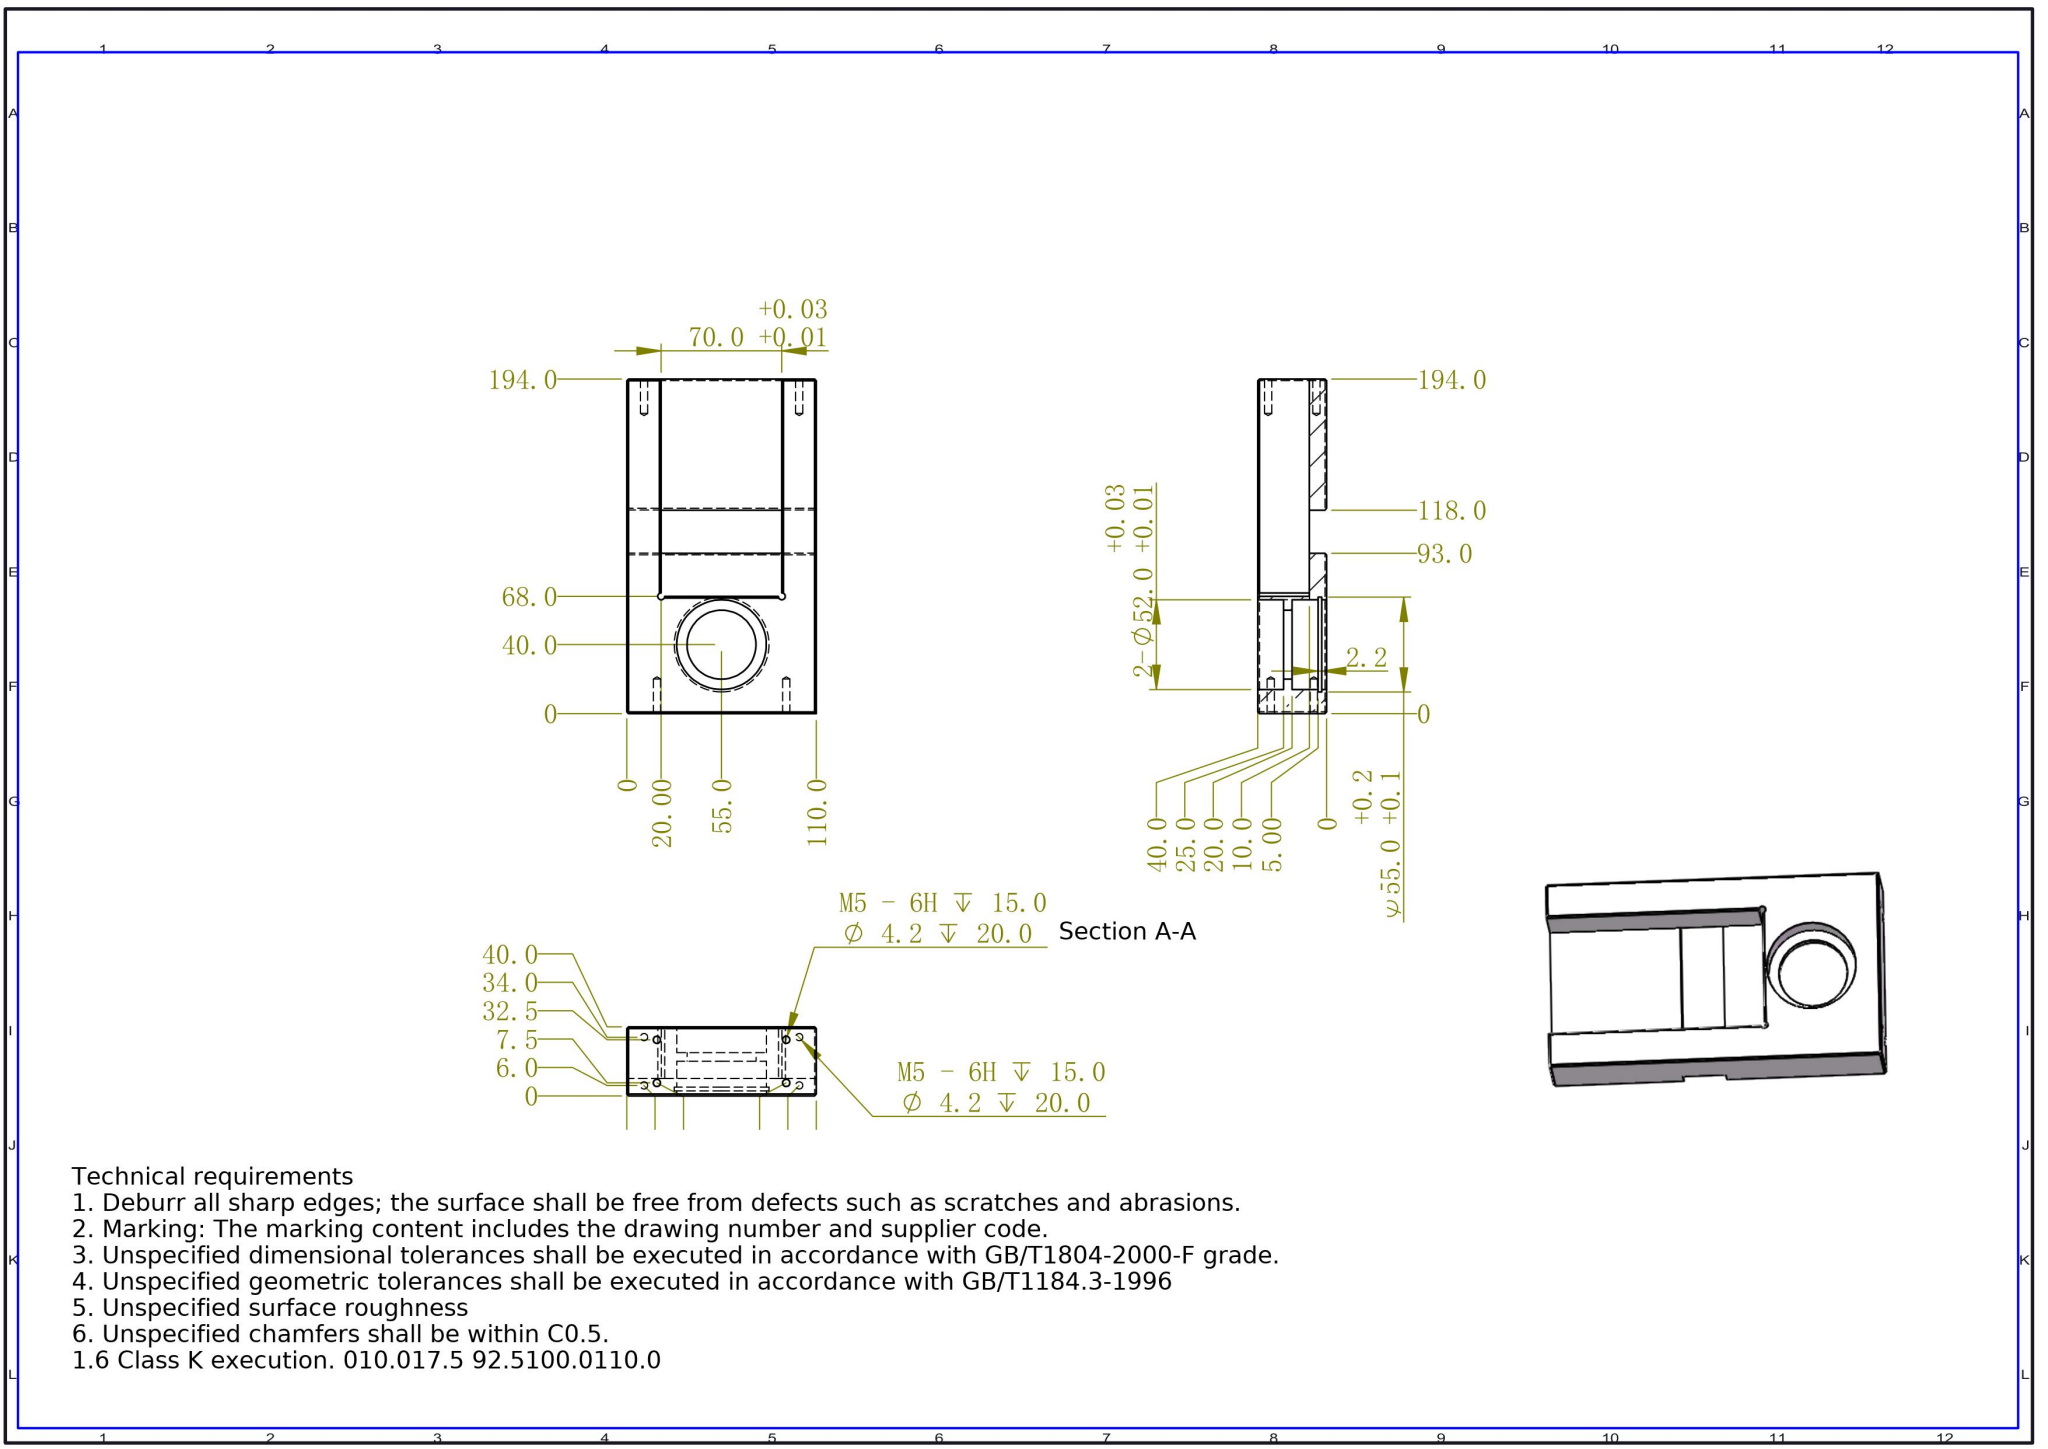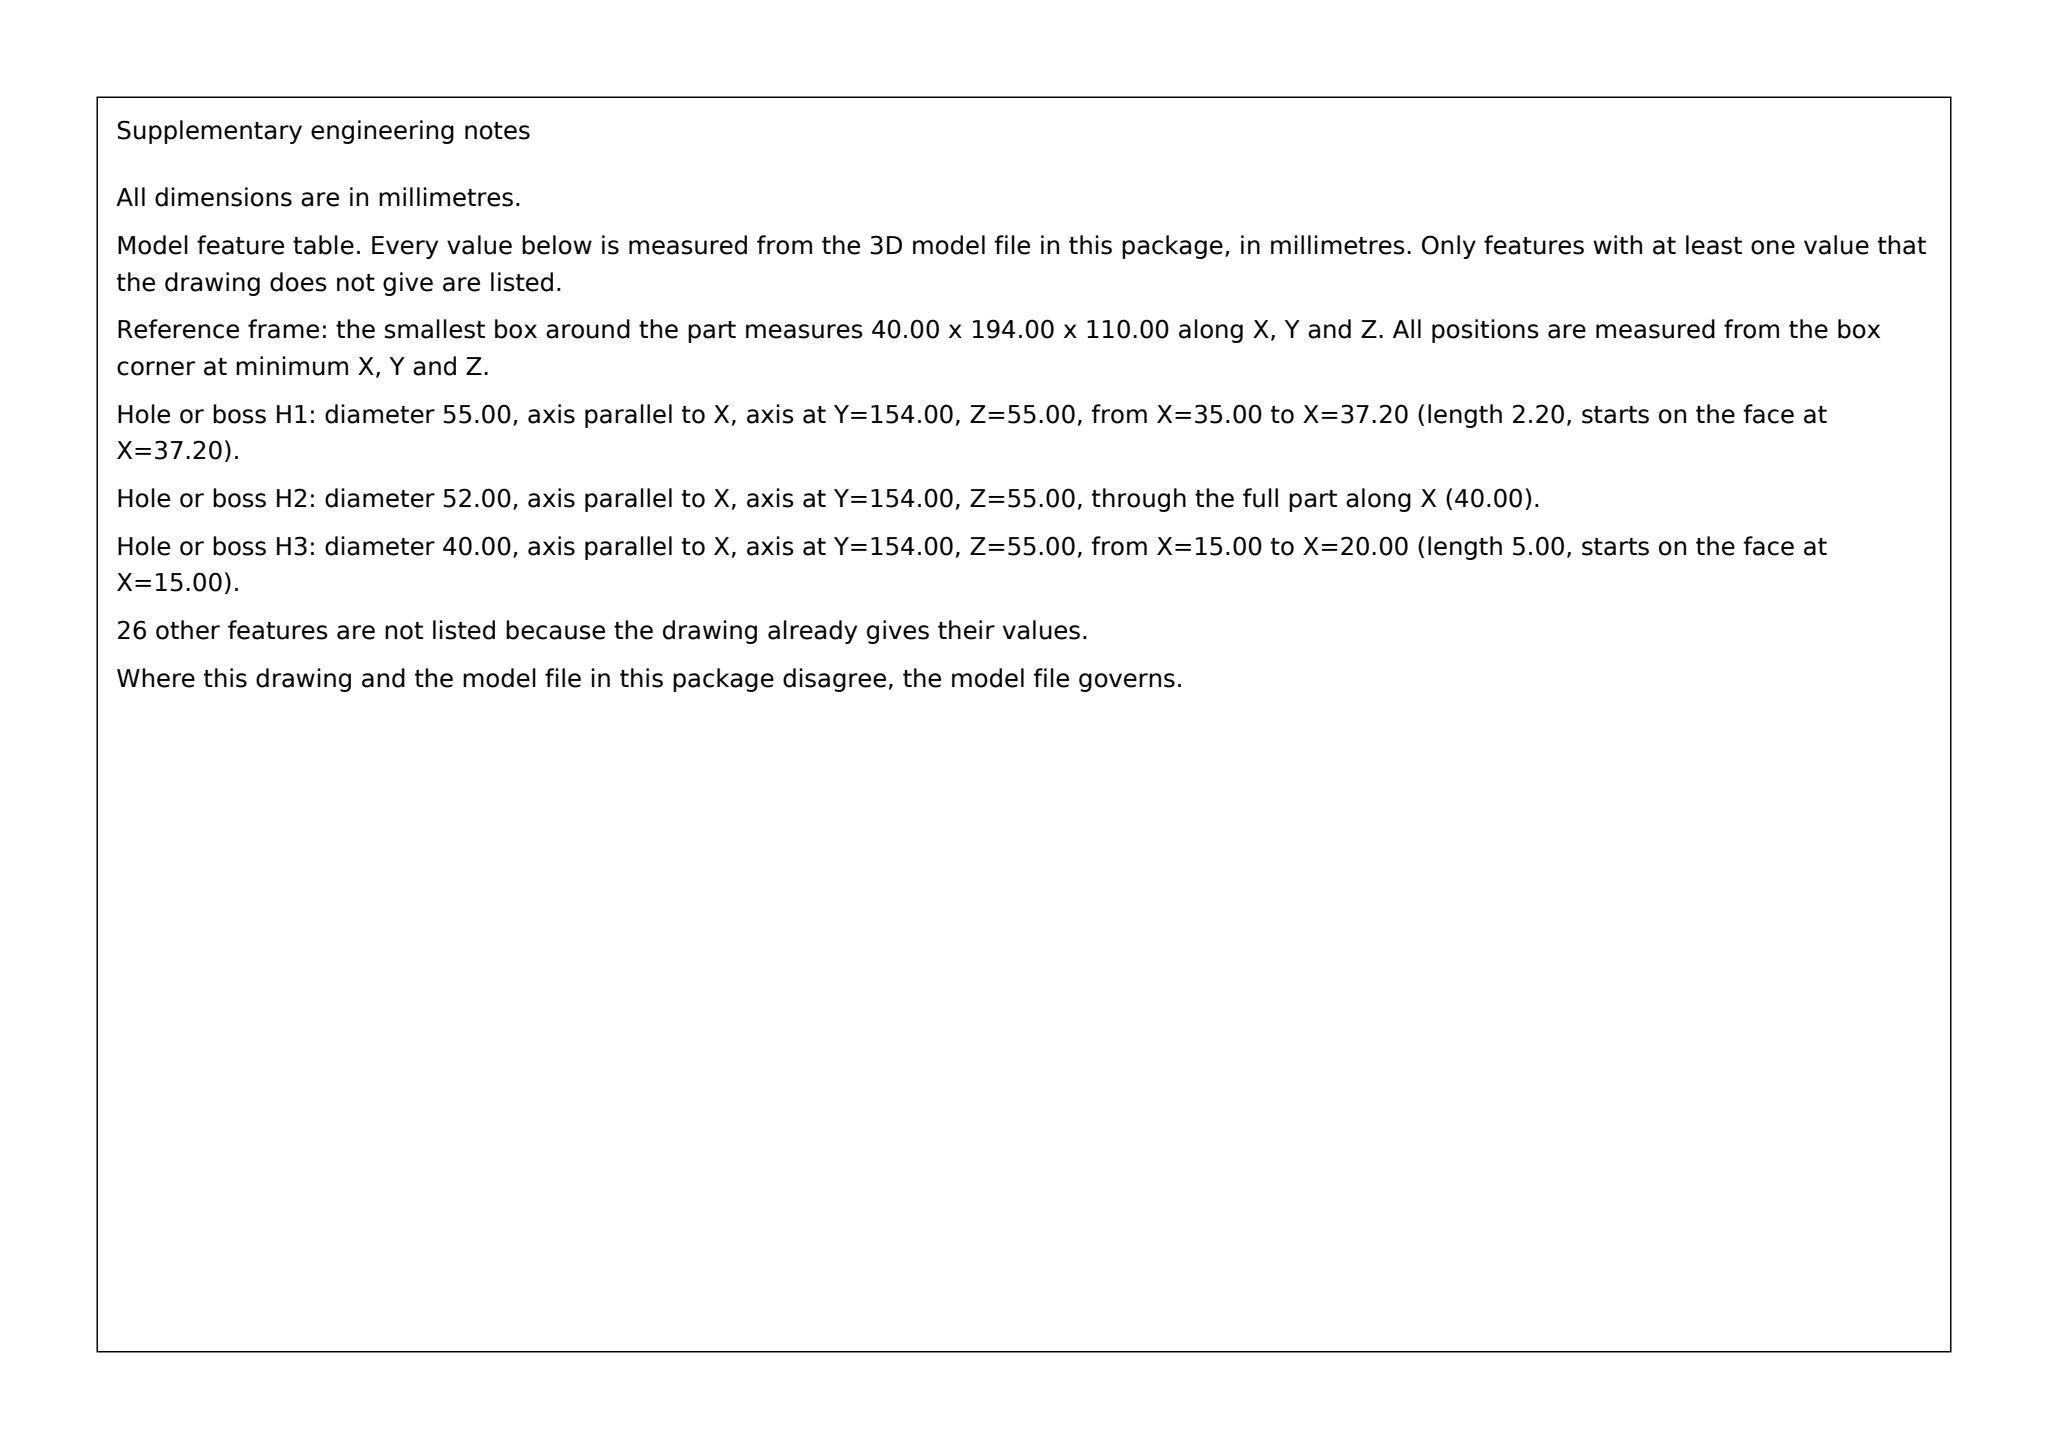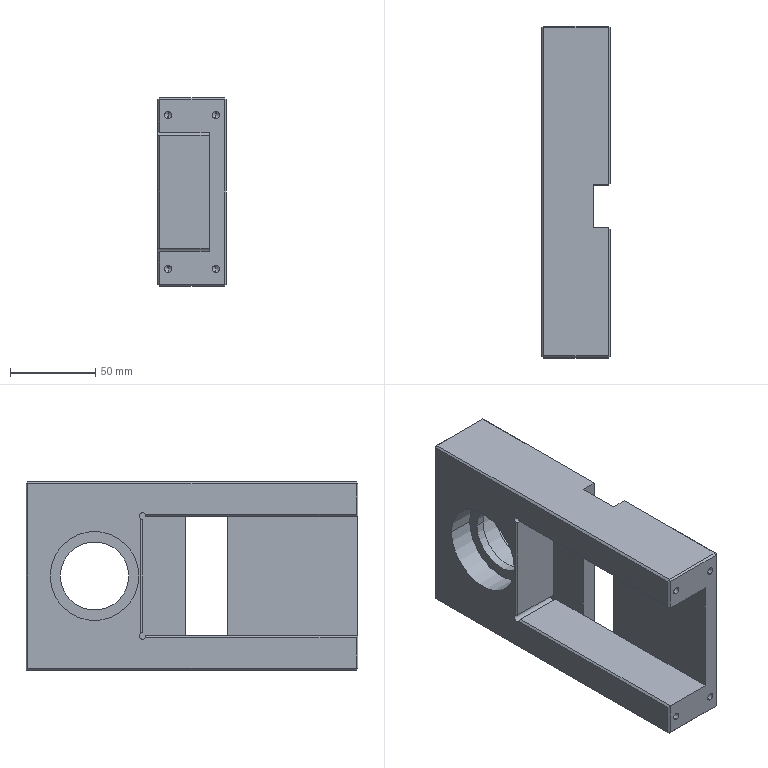Part | SolidWorks | mm | 1 solid | 89 faces | box 40 x 194 x 110 mm | volume 476635 mm3 | plane 45 | cylinder 28 | cone 16 | commonest cylinder face diameters 4.2 x16 52 x6 55 x2 40 x2 4 x2
build123d program:
from build123d import *

# Parameters (mm, degrees)
SKETCH1_W             = 40
SKETCH1_H             = 194
BOSS_EXTRUDE1_DEPTH   = 55
SKETCH2_W             = 70
SKETCH2_H             = 126
CUT_EXTRUDE1_DEPTH    = 30
SKETCH3_W             = 110
SKETCH3_H             = 25
CUT_EXTRUDE2_DEPTH    = 10
SKETCH4_R             = 20
CUT_EXTRUDE3_DEPTH    = 101
SKETCH5_R             = 26
CUT_EXTRUDE4_DEPTH    = 15
CUT_EXTRUDE5_START    = -20
SKETCH6_R             = 26
CUT_EXTRUDE5_DEPTH    = 20
CUT_EXTRUDE6_START    = -5
SKETCH7_R             = 27.5
SKETCH7_R_2           = 26
CUT_EXTRUDE6_DEPTH    = 2.2
M5_TAPPED_HOLE1_D     = 4.2
M5_TAPPED_HOLE1_DEPTH = 20
M5_TAPPED_HOLE1_TIP   = 1.262
CHAMFER1_SIZE         = 1
SKETCH11_R            = 2
CUT_EXTRUDE7_DEPTH    = 30
M5_TAPPED_HOLE2_D     = 4.2
M5_TAPPED_HOLE2_DEPTH = 20
M5_TAPPED_HOLE2_TIP   = 1.262


with BuildPart() as part:
    # Sketch1 → Boss-Extrude1 (new, symmetric)
    with BuildSketch(Plane.XY):
        Rectangle(SKETCH1_W, SKETCH1_H)
    extrude(amount=BOSS_EXTRUDE1_DEPTH, both=True)

    # Sketch2 → Cut-Extrude1 (cut)
    with BuildSketch(Plane.ZY.offset(20)):
        with Locations((0, -34)):
            Rectangle(SKETCH2_W, SKETCH2_H)
    extrude(amount=-CUT_EXTRUDE1_DEPTH, mode=Mode.SUBTRACT)

    # Sketch3 → Cut-Extrude2 (cut)
    with BuildSketch(Plane(origin=(20, 0, 0), x_dir=(0, 0, -1), z_dir=(1, 0, 0))):
        with Locations((0, -8.5)):
            Rectangle(SKETCH3_W, SKETCH3_H)
    extrude(amount=-CUT_EXTRUDE2_DEPTH, mode=Mode.SUBTRACT)

    # Sketch4 → Cut-Extrude3 (cut)
    with BuildSketch(Plane(origin=(20, 0, 0), x_dir=(0, 0, -1), z_dir=(1, 0, 0))):
        with Locations(Location((0, 57, 0), (0, 0, 90))):
            Circle(SKETCH4_R)
    extrude(amount=-CUT_EXTRUDE3_DEPTH, mode=Mode.SUBTRACT)

    # Sketch5 → Cut-Extrude4 (cut)
    with BuildSketch(Plane.ZY.offset(20)):
        with Locations(Location((0, 57, 0), (0, 0, 270))):
            Circle(SKETCH5_R)
    extrude(amount=-CUT_EXTRUDE4_DEPTH, mode=Mode.SUBTRACT)

    # Sketch6 → Cut-Extrude5 (cut)
    with BuildSketch(Plane(origin=(20, 0, 0), x_dir=(0, 0, -1), z_dir=(1, 0, 0)).offset(CUT_EXTRUDE5_START)):
        with Locations(Location((0, 57, 0), (0, 0, 270))):
            Circle(SKETCH6_R)
    extrude(amount=CUT_EXTRUDE5_DEPTH, mode=Mode.SUBTRACT)

    # Sketch7 → Cut-Extrude6 (cut)
    with BuildSketch(Plane(origin=(20, 0, 0), x_dir=(0, 0, -1), z_dir=(1, 0, 0)).offset(CUT_EXTRUDE6_START)):
        with Locations(Location((0, 57, 0), (0, 0, 90))):
            Circle(SKETCH7_R)
        with Locations(Location((0, 57, 0), (0, 0, 90))):
            Circle(SKETCH7_R_2, mode=Mode.SUBTRACT)
    extrude(amount=CUT_EXTRUDE6_DEPTH, mode=Mode.SUBTRACT)

    # M5 Tapped Hole1
    with Locations(Plane(origin=(0, -97, 0), x_dir=(-1, 0, 0), z_dir=(0, -1, 0))):
        with Locations((14, -45), (-14, -45), (-14, 45), (14, 45)):
            Hole(M5_TAPPED_HOLE1_D / 2, depth=M5_TAPPED_HOLE1_DEPTH)
            with Locations((0, 0, -(M5_TAPPED_HOLE1_DEPTH + M5_TAPPED_HOLE1_TIP / 2))):  # 118° drill point
                Cone(0, M5_TAPPED_HOLE1_D / 2, M5_TAPPED_HOLE1_TIP, mode=Mode.SUBTRACT)

    # Chamfer1
    chamfer1_edges = [part.edges().sort_by_distance(p)[0] for p in [
        (20, -59, 55),
        (-20, -97, -45),
        (0, 97, 55),
        (-20, -34, -35),
        (-20, -34, 35),
        (-20, 29, 0),
        (20, 50.5, -55),
        (20, 50.5, 55),
        (20, -21, 0),
        (20, 4, 0),
        (-20, 0, 55),
        (20, -59, -55),
        (0, -97, -55),
        (-20, 0, -55),
        (-20, 97, 0),
        (20, 97, 0),
        (20, -97, 0),
        (-20, -97, 45),
        (0, -97, 55),
    ]]
    chamfer(chamfer1_edges, length=CHAMFER1_SIZE)

    # Sketch11 → Cut-Extrude7 (cut)
    with BuildSketch(Plane.ZY.offset(20)):
        with Locations((-35, 29)):
            Circle(SKETCH11_R)
        with Locations((35, 29)):
            Circle(SKETCH11_R)
    extrude(amount=-CUT_EXTRUDE7_DEPTH, mode=Mode.SUBTRACT)

    # M5 Tapped Hole2
    with Locations(Plane(origin=(0, 97, 0), x_dir=(1, 0, 0), z_dir=(0, 1, 0))):
        with Locations((-12.5, -37.5), (12.5, -37.5), (12.5, 37.5), (-12.5, 37.5)):
            Hole(M5_TAPPED_HOLE2_D / 2, depth=M5_TAPPED_HOLE2_DEPTH)
            with Locations((0, 0, -(M5_TAPPED_HOLE2_DEPTH + M5_TAPPED_HOLE2_TIP / 2))):  # 118° drill point
                Cone(0, M5_TAPPED_HOLE2_D / 2, M5_TAPPED_HOLE2_TIP, mode=Mode.SUBTRACT)


solid = part.part